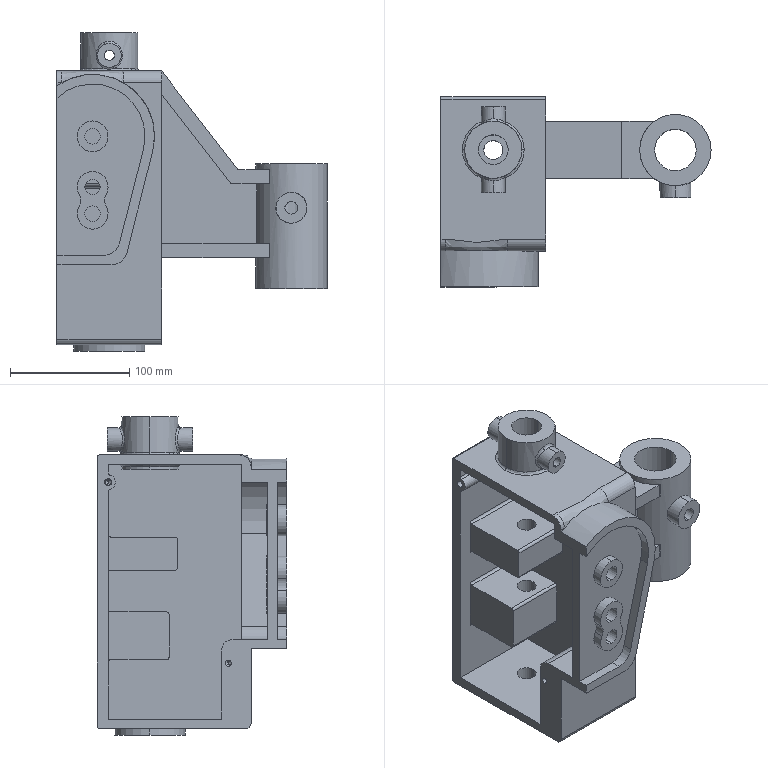Component | SolidWorks | 8-2 | 1 solid | 163 faces | volume 1492334 mm3 | cylinder 83 | plane 67 | cone 6 | spline 5 | torus 2 | commonest cylinder face diameters 26 x12 4 x12 20 x11 13 x6 16 x6 5 x4 48 x4 8.5 x4